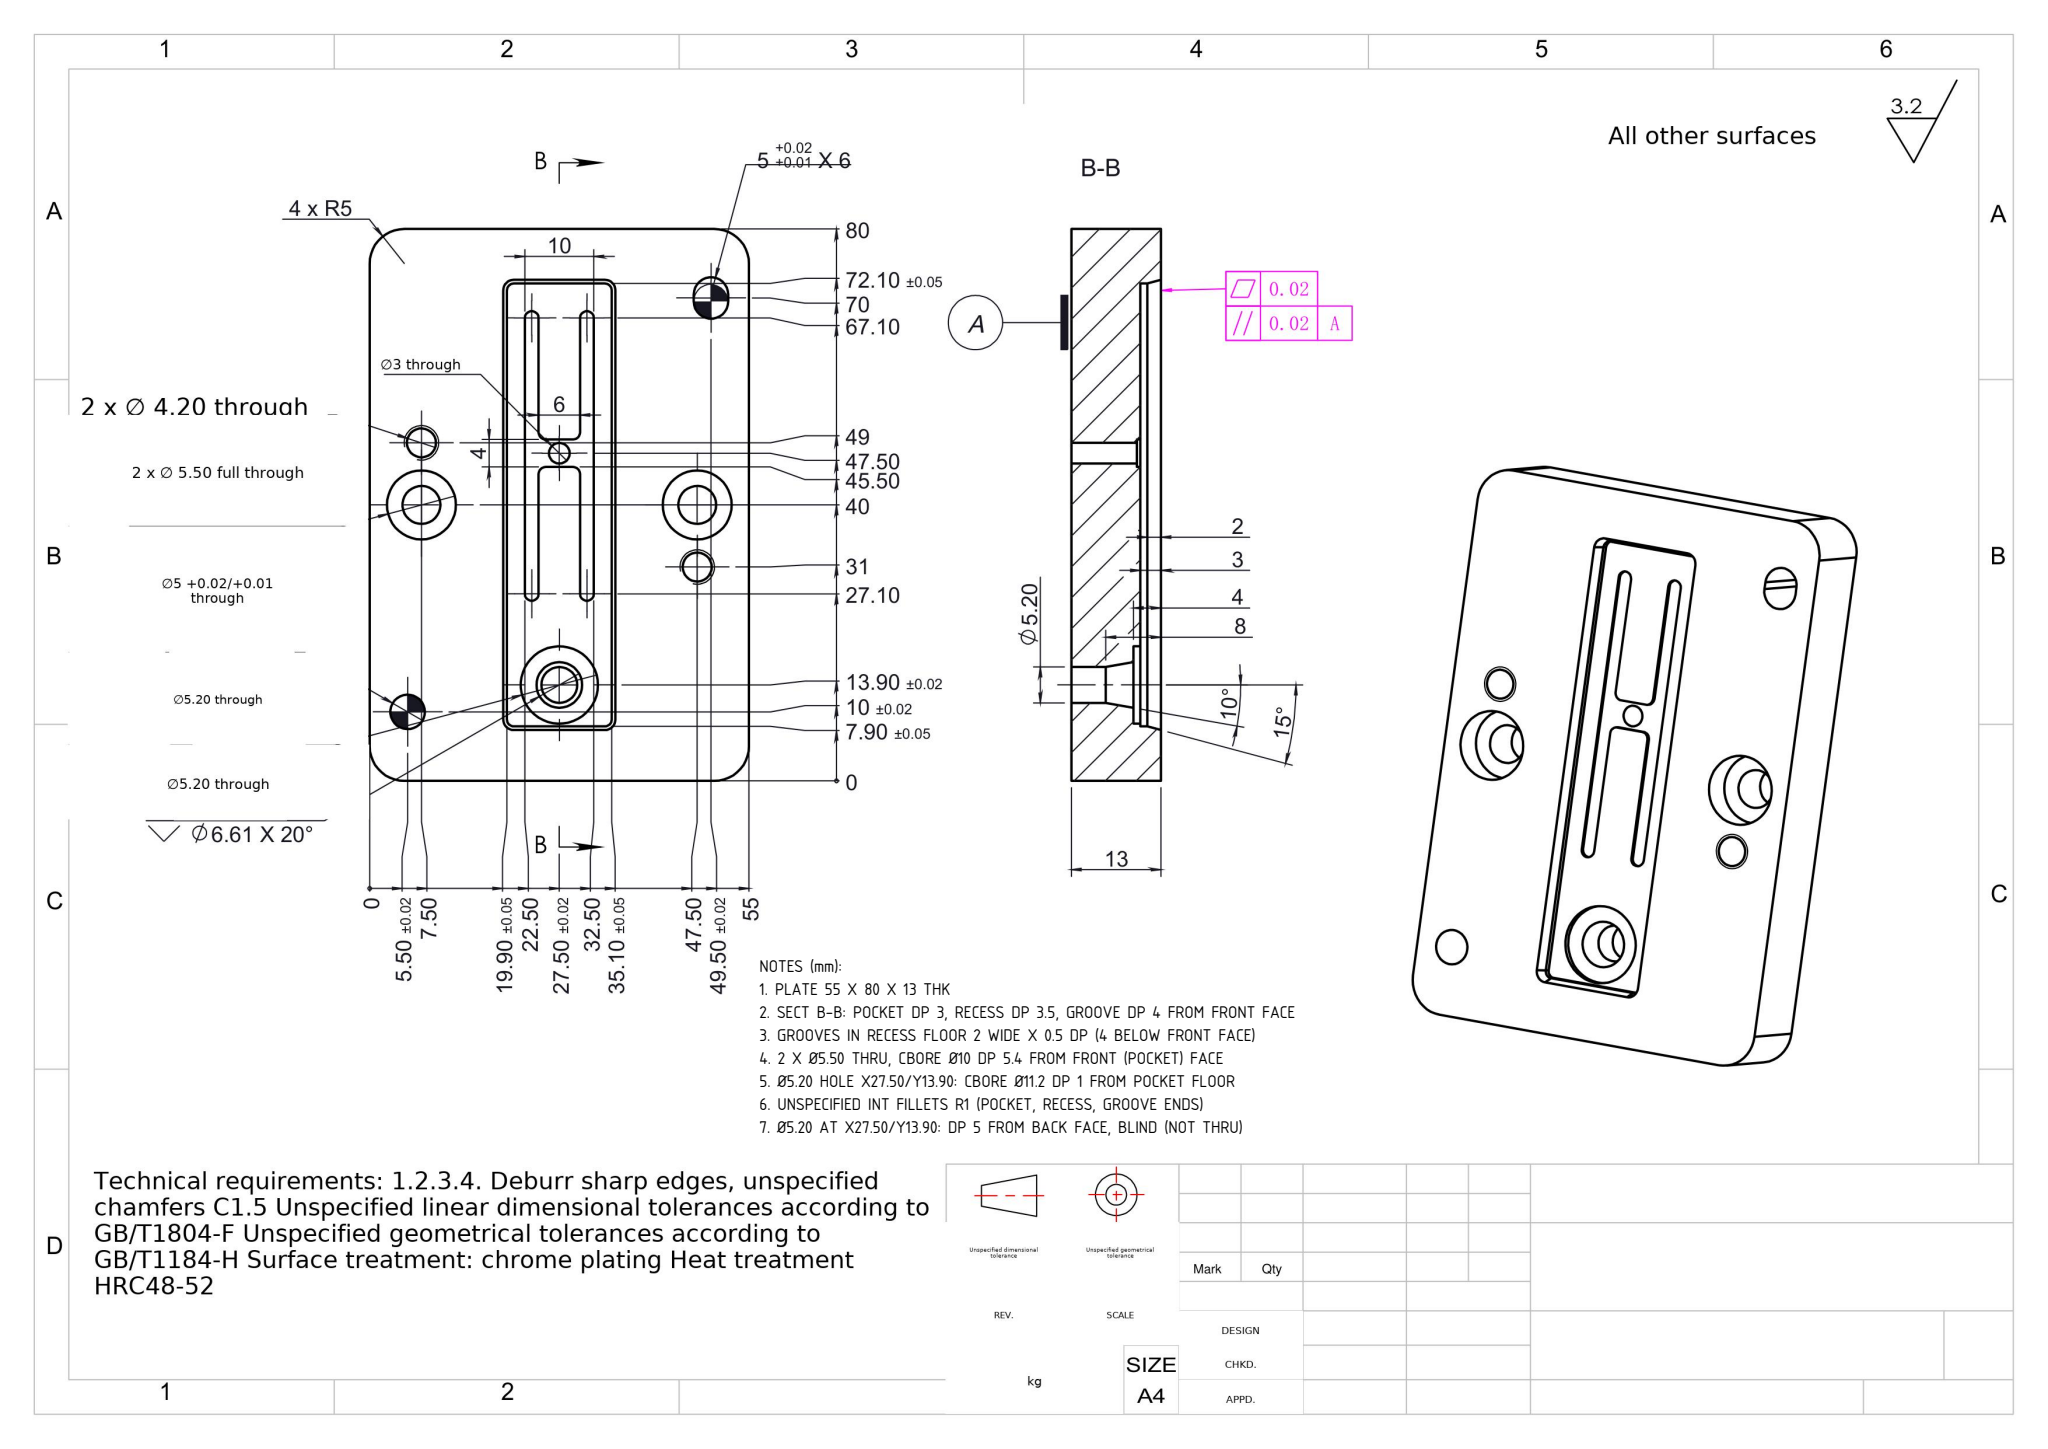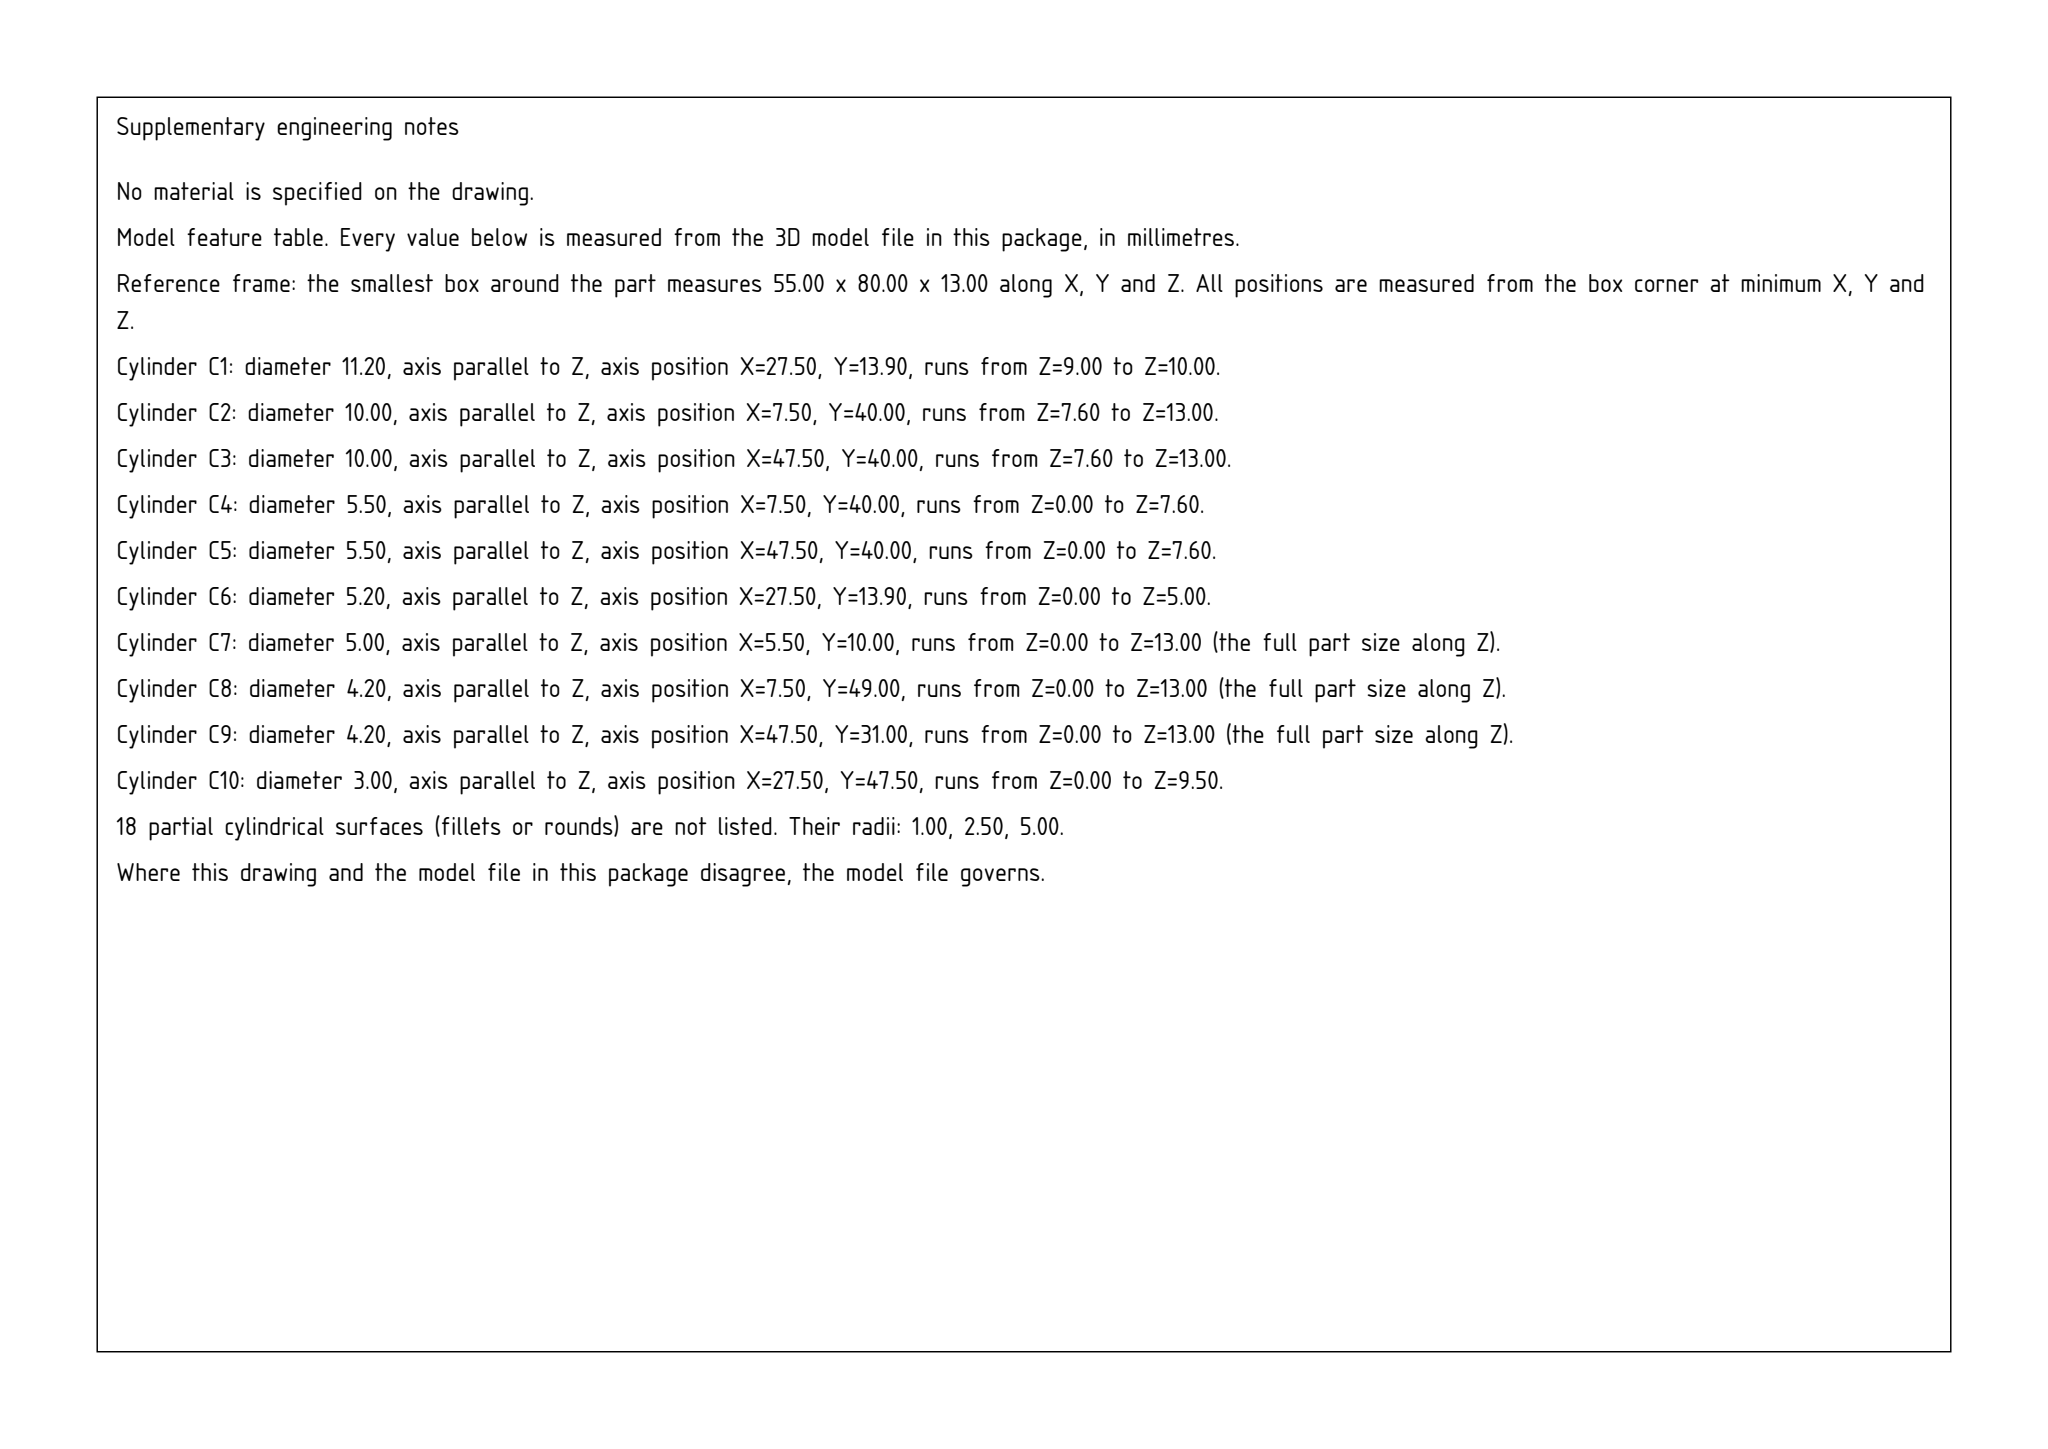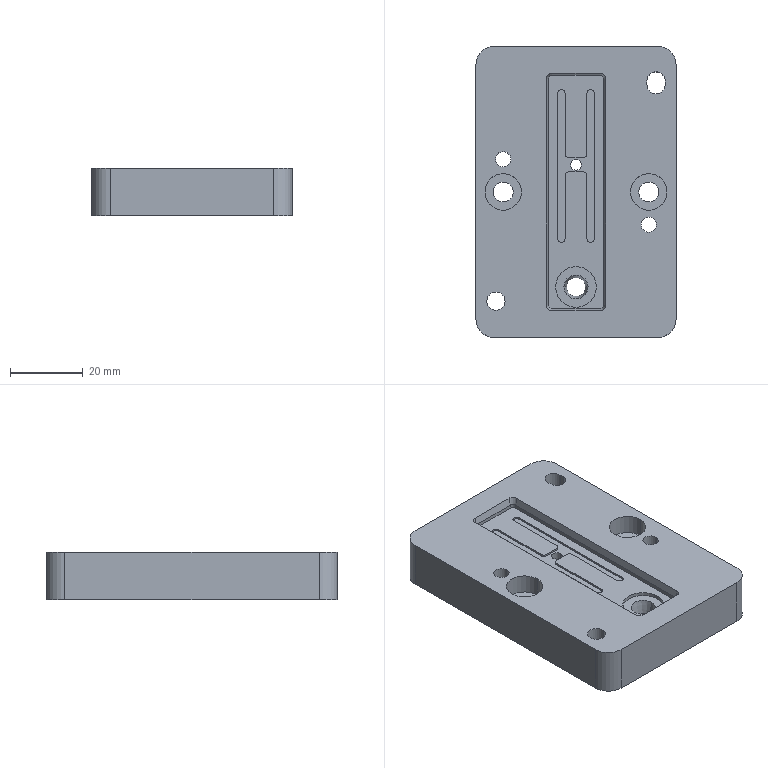Part | SolidWorks | mm | 1 solid | 73 faces | box 55 x 80 x 13 mm | volume 51289 mm3 | cylinder 38 | plane 29 | cone 6 | commonest cylinder face diameters 2 x12 10 x8 4.2 x4 5.5 x4 5 x4 3 x2 11.2 x2 5.2 x2
Drawing notes:
PLATE 55 X 80 X 13 THK | from the solid: bbox_xyz 55.0 x 80.0 x 13.0
SECT B-B: POCKET DP 3, RECESS DP 3.5, GROOVE DP 4 FROM FRONT FACE | from the solid: z planes 13.0 (front face), 10.0, 9.5, 9.0
GROOVES IN RECESS FLOOR 2 WIDE X 0.5 DP (4 BELOW FRONT FACE) | from the solid: Ø2 cyls len 0.5 at y44.5/50.5 and 27.1/67.1; z planes 9.5 floor, 9.0 bottom
2 X Ø5.50 THRU, CBORE Ø10 DP 5.4 FROM FRONT (POCKET) FACE | from the solid: cyl Ø10 z len 5.4 at (7.5,40) & (47.5,40); Ø5.5 len 7.6 from z0; front face z=13
Ø5.20 HOLE X27.50/Y13.90: CBORE Ø11.2 DP 1 FROM POCKET FLOOR | from the solid: cyl Ø11.2 z len 1.0 at (27.5,13.9); pocket floor z=10, recess bottom z=9.0
UNSPECIFIED INT FILLETS R1 (POCKET, RECESS, GROOVE ENDS) | from the solid: Ø2 corner cyls at 20.9/34.1 x 8.9/71.1, 23.5/31.5 x 27.1/67.1, 25.5/29.5 x 44.5/50.5
Ø5.20 AT X27.50/Y13.90: DP 5 FROM BACK FACE, BLIND (NOT THRU) | from the solid: cyl [5.2,z,[27.5,13.9],len 5.0] + cbore [11.2,z,[27.5,13.9],len 1.0]; plate 13 thk, floor 8 below front face
build123d program:
from build123d import *
from OCP.BRepFilletAPI import BRepFilletAPI_MakeChamfer

# Parameters (mm, degrees)
SKETCH1_W                                       = 55
SKETCH1_H                                       = 80
BOSS_EXTRUDE1_DEPTH                             = 13
SKETCH4_W                                       = 15.2
SKETCH4_H                                       = 64.2
CUT_EXTRUDE1_DEPTH                              = 3
SKETCH6_R                                       = 2.6
CUT_EXTRUDE3_DEPTH                              = 50.561
FILLET5_R                                       = 5
SKETCH11_R                                      = 2.5
CUT_EXTRUDE4_DEPTH                              = 51.252
M5_HEX_SOCKET_HEAD_CAP_SCREW_CBORE1_D           = 5.5
M5_HEX_SOCKET_HEAD_CAP_SCREW_CBORE1_CBORE_D     = 10
M5_HEX_SOCKET_HEAD_CAP_SCREW_CBORE1_CBORE_DEPTH = 5.4
M5_TAPPED_HOLE2_D                               = 4.2
SKETCH17_R                                      = 5.6
CUT_EXTRUDE5_DEPTH                              = 1
CHAMFER1_SIZE                                   = 4
CHAMFER1_SIZE2                                  = 0.7053
FILLET6_R                                       = 1
CHAMFER2_SIZE                                   = 2
CHAMFER2_SIZE2                                  = 0.5359
CUT_EXTRUDE6_DEPTH                              = 0.5
SKETCH19_W                                      = 6
SKETCH19_H                                      = 4
CUT_EXTRUDE7_DEPTH                              = 0.5
FILLET7_R                                       = 1
SKETCH20_R                                      = 1.5
CUT_EXTRUDE8_DEPTH                              = 50.462


with BuildPart() as part:
    # Sketch1 → Boss-Extrude1 (new body)
    with BuildSketch(Plane.XY):
        Rectangle(SKETCH1_W, SKETCH1_H)
    extrude(amount=BOSS_EXTRUDE1_DEPTH)

    # Sketch4 → Cut-Extrude1 (cut)
    with BuildSketch(Plane.XY.offset(13)):
        Rectangle(SKETCH4_W, SKETCH4_H)
    extrude(amount=-CUT_EXTRUDE1_DEPTH, mode=Mode.SUBTRACT)

    # Sketch6 → Cut-Extrude3 (cut, through all)
    with BuildSketch(Plane.XY.offset(10)):
        with Locations((0, -26.1)):
            Circle(SKETCH6_R)
    extrude(amount=-CUT_EXTRUDE3_DEPTH, mode=Mode.SUBTRACT)

    # Fillet5
    fillet5_edges = [part.edges().sort_by_distance(p)[0] for p in [
        (27.5, -40, 6.5),
        (-27.5, -40, 6.5),
        (-27.5, 40, 6.5),
        (27.5, 40, 6.5),
    ]]
    fillet(fillet5_edges, radius=FILLET5_R)

    # Sketch11 → Cut-Extrude4 (cut, through all)
    with BuildSketch(Plane.XY.offset(13)):
        with Locations((-22, -30)):
            Circle(SKETCH11_R)
        with BuildLine():
            Line((24.5, 30.5), (24.5, 29.5))
            ThreePointArc((24.5, 29.5), (22, 27), (19.5, 29.5))
            Line((19.5, 29.5), (19.5, 30.5))
            ThreePointArc((19.5, 30.5), (22, 33), (24.5, 30.5))
        make_face()
    extrude(amount=-CUT_EXTRUDE4_DEPTH, mode=Mode.SUBTRACT)

    # M5 Hex Socket Head Cap Screw CBORE1 (through all)
    with Locations(Plane.XY.offset(13)):
        with Locations((-20, 0), (20, 0)):
            CounterBoreHole(M5_HEX_SOCKET_HEAD_CAP_SCREW_CBORE1_D / 2, M5_HEX_SOCKET_HEAD_CAP_SCREW_CBORE1_CBORE_D / 2, M5_HEX_SOCKET_HEAD_CAP_SCREW_CBORE1_CBORE_DEPTH)

    # M5 Tapped Hole2 (through all)
    with Locations(Plane.XY.offset(13)):
        with Locations((-20, 9), (20, -9)):
            Hole(M5_TAPPED_HOLE2_D / 2)

    # Sketch17 → Cut-Extrude5 (cut)
    with BuildSketch(Plane.XY.offset(10)):
        with Locations((0, -26.1)):
            Circle(SKETCH17_R)
    extrude(amount=-CUT_EXTRUDE5_DEPTH, mode=Mode.SUBTRACT)

    # Chamfer1
    chamfer1_edges = [part.edges().sort_by_distance(p)[0] for p in [
        (-2.6, -26.1, 9),
    ]]
    chamfer1_side = [part.faces().sort_by_distance(p)[0] for p in [
        (-2.6, -26.1, 4.5),
    ]]
    chamfer(chamfer1_edges, length=CHAMFER1_SIZE, length2=CHAMFER1_SIZE2, reference=chamfer1_side[0])

    # Fillet6
    fillet6_edges = [part.edges().sort_by_distance(p)[0] for p in [
        (-7.6, -32.1, 11.5),
        (-7.6, 32.1, 11.5),
        (7.6, 32.1, 11.5),
        (7.6, -32.1, 11.5),
    ]]
    fillet(fillet6_edges, radius=FILLET6_R)

    # Chamfer2: one chamfer whose edges measure the first distance from different faces: ONE call of the kernel's chamfer builder (chamfer() names one face for all edges)
    chamfer2_edges_1 = [part.edges().sort_by_distance(p)[0] for p in [
        (0, -32.1, 13),
    ]]
    chamfer2_side_1 = [part.faces().sort_by_distance(p)[0] for p in [
        (0, -32.1, 11.5),
    ]]
    chamfer2_edges_2 = [part.edges().sort_by_distance(p)[0] for p in [
        (-7.6, 0, 13),
    ]]
    chamfer2_side_2 = [part.faces().sort_by_distance(p)[0] for p in [
        (-7.6, 0, 11.5),
    ]]
    chamfer2_edges_3 = [part.edges().sort_by_distance(p)[0] for p in [
        (7.6, 0, 13),
    ]]
    chamfer2_side_3 = [part.faces().sort_by_distance(p)[0] for p in [
        (7.6, 0, 11.5),
    ]]
    chamfer2_edges_4 = [part.edges().sort_by_distance(p)[0] for p in [
        (0, 32.1, 13),
    ]]
    chamfer2_side_4 = [part.faces().sort_by_distance(p)[0] for p in [
        (0, 32.1, 11.5),
    ]]
    chamfer2_edges_5 = [part.edges().sort_by_distance(p)[0] for p in [
        (-7.307, -31.807, 13),
    ]]
    chamfer2_side_5 = [part.faces().sort_by_distance(p)[0] for p in [
        (-7.307, -31.807, 11.5),
    ]]
    chamfer2_edges_6 = [part.edges().sort_by_distance(p)[0] for p in [
        (7.307, -31.807, 13),
    ]]
    chamfer2_side_6 = [part.faces().sort_by_distance(p)[0] for p in [
        (7.307, -31.807, 11.5),
    ]]
    chamfer2_edges_7 = [part.edges().sort_by_distance(p)[0] for p in [
        (7.307, 31.807, 13),
    ]]
    chamfer2_side_7 = [part.faces().sort_by_distance(p)[0] for p in [
        (7.307, 31.807, 11.5),
    ]]
    chamfer2_edges_8 = [part.edges().sort_by_distance(p)[0] for p in [
        (-7.307, 31.807, 13),
    ]]
    chamfer2_side_8 = [part.faces().sort_by_distance(p)[0] for p in [
        (-7.307, 31.807, 11.5),
    ]]
    chamfer2 = BRepFilletAPI_MakeChamfer(part.part.solid().wrapped)
    for e in chamfer2_edges_1:
        chamfer2.Add(CHAMFER2_SIZE, CHAMFER2_SIZE2, e.wrapped, chamfer2_side_1[0].wrapped)  # the first distance lies on this face
    for e in chamfer2_edges_2:
        chamfer2.Add(CHAMFER2_SIZE, CHAMFER2_SIZE2, e.wrapped, chamfer2_side_2[0].wrapped)  # the first distance lies on this face
    for e in chamfer2_edges_3:
        chamfer2.Add(CHAMFER2_SIZE, CHAMFER2_SIZE2, e.wrapped, chamfer2_side_3[0].wrapped)  # the first distance lies on this face
    for e in chamfer2_edges_4:
        chamfer2.Add(CHAMFER2_SIZE, CHAMFER2_SIZE2, e.wrapped, chamfer2_side_4[0].wrapped)  # the first distance lies on this face
    for e in chamfer2_edges_5:
        chamfer2.Add(CHAMFER2_SIZE, CHAMFER2_SIZE2, e.wrapped, chamfer2_side_5[0].wrapped)  # the first distance lies on this face
    for e in chamfer2_edges_6:
        chamfer2.Add(CHAMFER2_SIZE, CHAMFER2_SIZE2, e.wrapped, chamfer2_side_6[0].wrapped)  # the first distance lies on this face
    for e in chamfer2_edges_7:
        chamfer2.Add(CHAMFER2_SIZE, CHAMFER2_SIZE2, e.wrapped, chamfer2_side_7[0].wrapped)  # the first distance lies on this face
    for e in chamfer2_edges_8:
        chamfer2.Add(CHAMFER2_SIZE, CHAMFER2_SIZE2, e.wrapped, chamfer2_side_8[0].wrapped)  # the first distance lies on this face
    add(Compound.cast(chamfer2.Shape()), mode=Mode.REPLACE)

    # Sketch18 → Cut-Extrude6 (cut)
    with BuildSketch(Plane.XY.offset(10)):
        with BuildLine():
            Line((5, 27.1), (5, -12.9))
            ThreePointArc((5, -12.9), (4, -13.9), (3, -12.9))
            Line((3, -12.9), (3, 27.1))
            ThreePointArc((3, 27.1), (4, 28.1), (5, 27.1))
        make_face()
        with BuildLine():
            Line((-5, 27.1), (-5, -12.9))
            ThreePointArc((-5, -12.9), (-4, -13.9), (-3, -12.9))
            Line((-3, -12.9), (-3, 27.1))
            ThreePointArc((-3, 27.1), (-4, 28.1), (-5, 27.1))
        make_face()
    extrude(amount=-CUT_EXTRUDE6_DEPTH, mode=Mode.SUBTRACT)

    # Sketch19 → Cut-Extrude7 (cut)
    with BuildSketch(Plane.XY.offset(10)):
        with Locations((0, 7.5)):
            Rectangle(SKETCH19_W, SKETCH19_H)
    extrude(amount=-CUT_EXTRUDE7_DEPTH, mode=Mode.SUBTRACT)

    # Fillet7
    fillet7_edges = [part.edges().sort_by_distance(p)[0] for p in [
        (-3, 5.5, 9.75),
        (-3, 9.5, 9.75),
        (3, 9.5, 9.75),
        (3, 5.5, 9.75),
    ]]
    fillet(fillet7_edges, radius=FILLET7_R)

    # Sketch20 → Cut-Extrude8 (cut, through all)
    with BuildSketch(Plane.XY.offset(9.5)):
        with Locations((0, 7.5)):
            Circle(SKETCH20_R)
    extrude(amount=-CUT_EXTRUDE8_DEPTH, mode=Mode.SUBTRACT)


solid = part.part